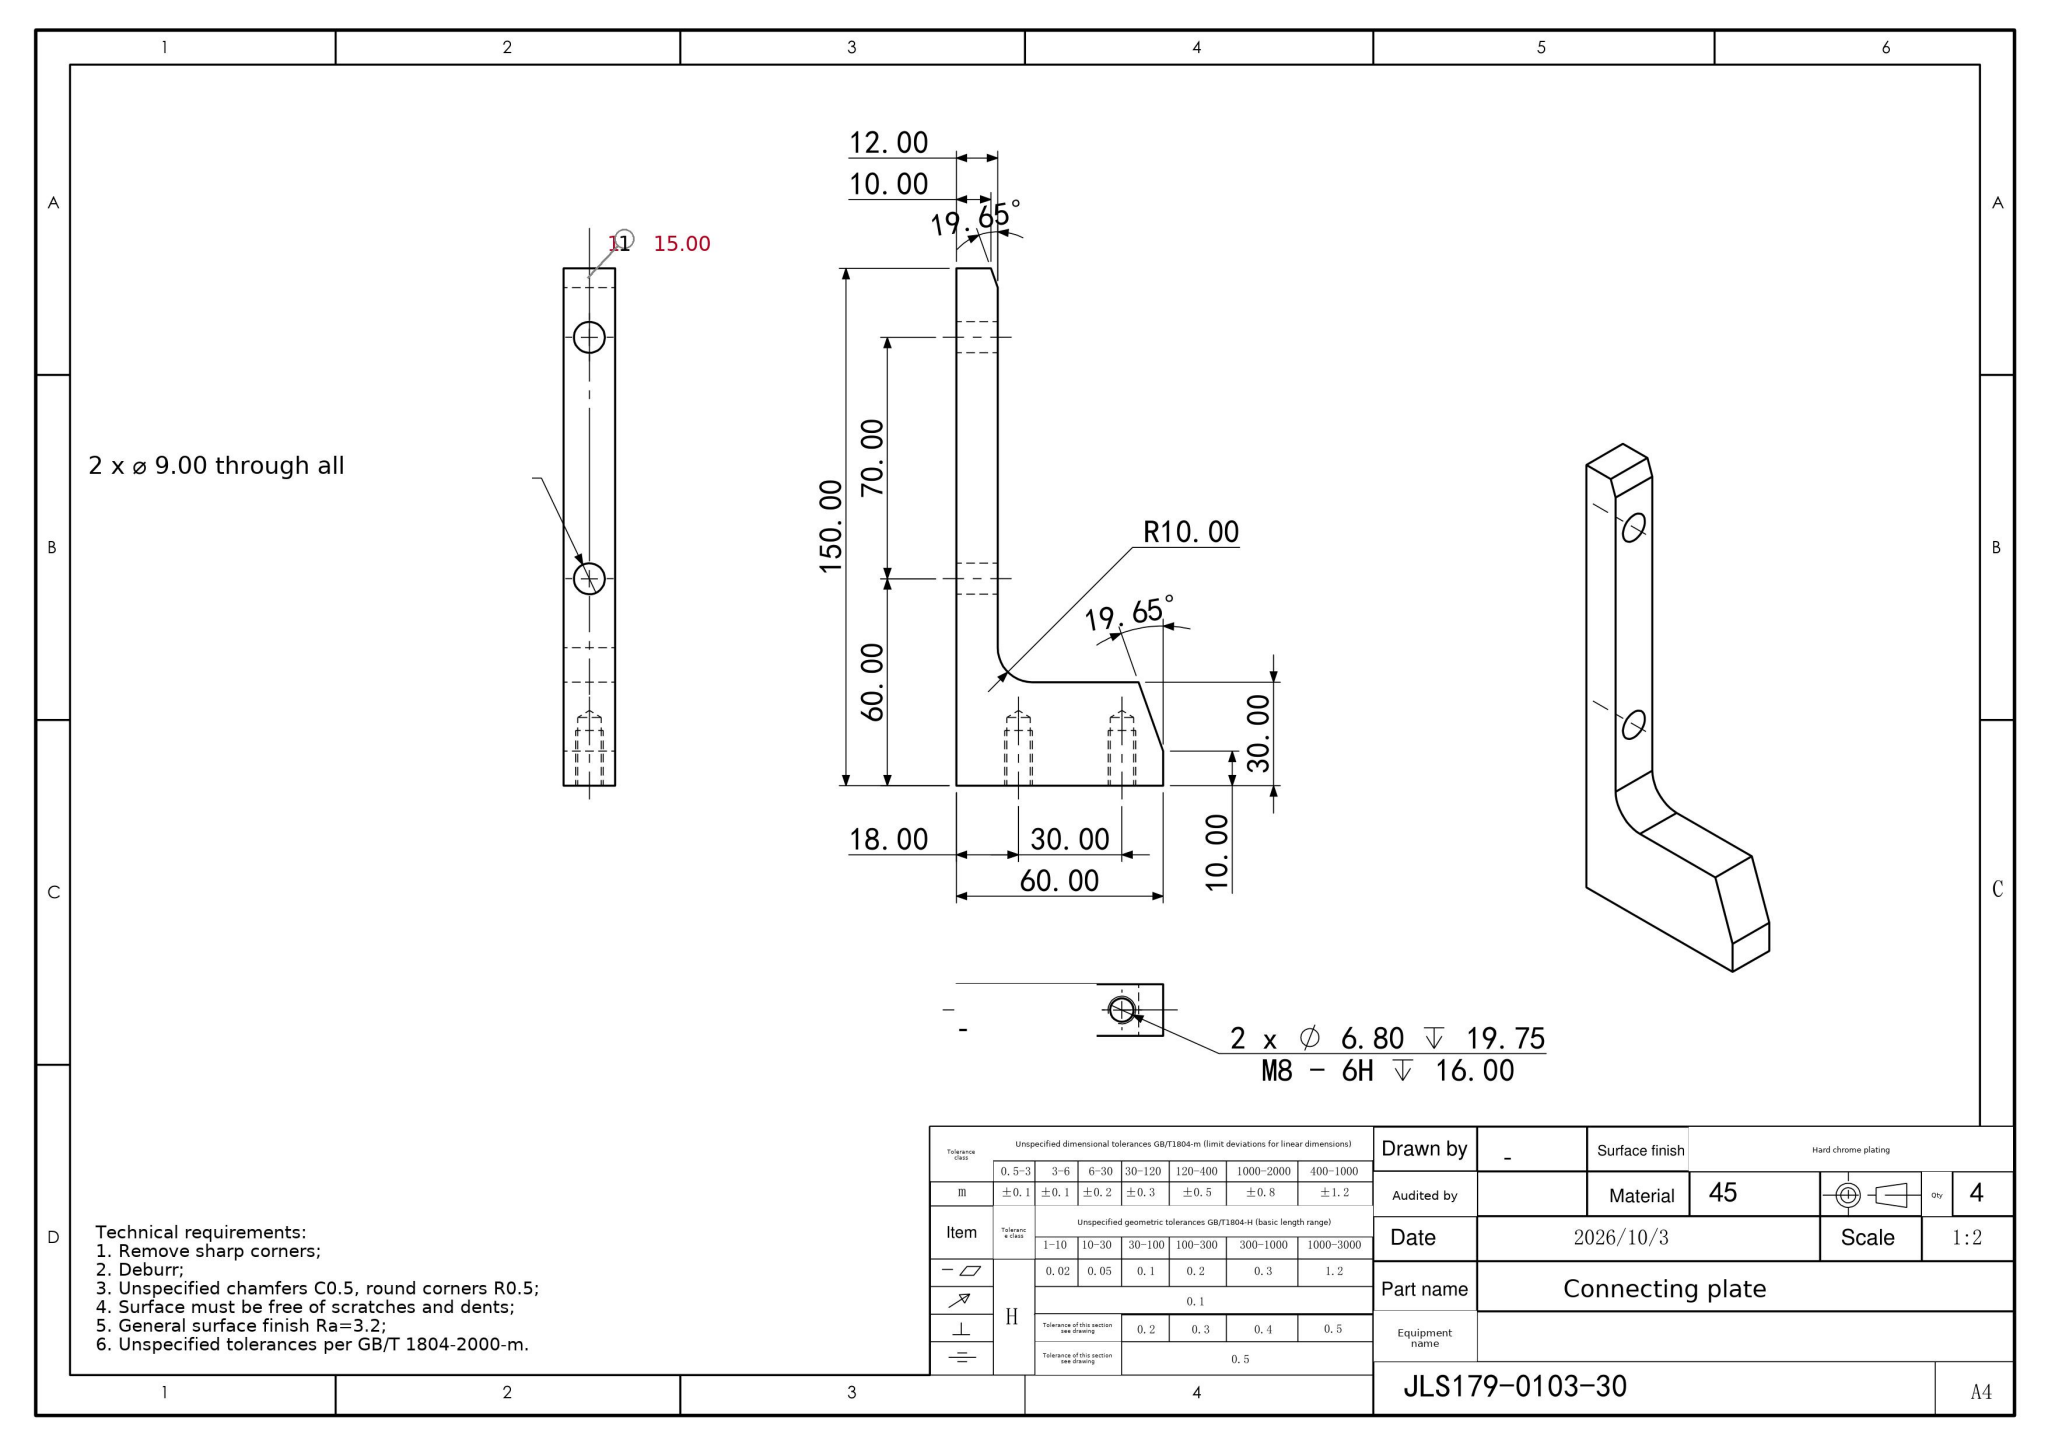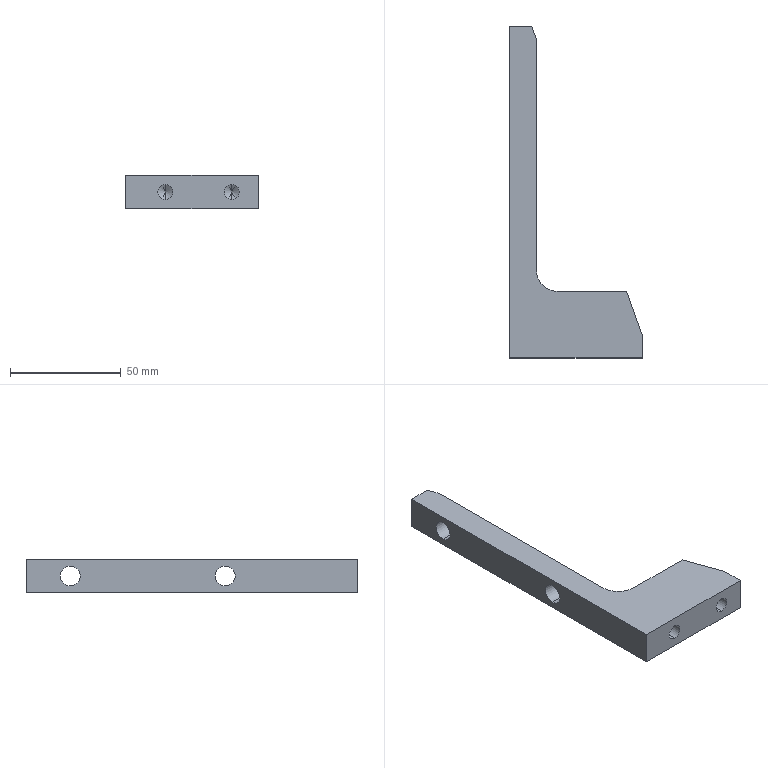Part | SolidWorks | mm | material 45 | 1 solid | 23 faces | box 60 x 150 x 15 mm | volume 44756 mm3 | plane 10 | cylinder 9 | cone 4 | commonest cylinder face diameters 6.8 x4 9 x4 20 x1
build123d program:
from build123d import *

# Parameters (mm, degrees)
BOSS_EXTRUDE1_DEPTH      = 7.5
F_9_0_9_DIAMETER_HOLE1_D = 9
M8_TAPPED_HOLE2_D        = 6.8
M8_TAPPED_HOLE2_DEPTH    = 19.75
M8_TAPPED_HOLE2_TIP      = 2.043
SKETCH6_W                = 90.036
SKETCH6_H                = 126.144
CUT_EXTRUDE1_DEPTH       = 163.25
FILLET1_R                = 10


with BuildPart() as part:
    # Sketch1 → Boss-Extrude1 (new, symmetric)
    with BuildSketch(Plane.XY):
        Polygon((0, 0), (0, 150), (10, 150), (60, 10), (60, 0), align=None)
    extrude(amount=BOSS_EXTRUDE1_DEPTH, both=True)

    # 9.0 _9_ Diameter Hole1 (through all)
    with Locations(Plane.ZY):
        with Locations((0, 130), (0, 60)):
            Hole(F_9_0_9_DIAMETER_HOLE1_D / 2)

    # M8 Tapped Hole2
    with Locations(Plane(origin=(0, 0, 0), x_dir=(-1, 0, 0), z_dir=(0, -1, 0))):
        with Locations((-48, 0), (-18, 0)):
            Hole(M8_TAPPED_HOLE2_D / 2, depth=M8_TAPPED_HOLE2_DEPTH)
            with Locations((0, 0, -(M8_TAPPED_HOLE2_DEPTH + M8_TAPPED_HOLE2_TIP / 2))):  # 118° drill point
                Cone(0, M8_TAPPED_HOLE2_D / 2, M8_TAPPED_HOLE2_TIP, mode=Mode.SUBTRACT)

    # Sketch6 → Cut-Extrude1 (cut, through all)
    with BuildSketch(Plane.XY.offset(7.5)):
        with Locations((57.018, 93.072)):
            Rectangle(SKETCH6_W, SKETCH6_H)
    extrude(amount=-CUT_EXTRUDE1_DEPTH, mode=Mode.SUBTRACT)

    # Fillet1
    fillet1_edges = [part.edges().sort_by_distance(p)[0] for p in [
        (12, 30, 0),
    ]]
    fillet(fillet1_edges, radius=FILLET1_R)


solid = part.part
STEP:
#1=CARTESIAN_POINT('',(48.,19.75,3.4));
#2=VERTEX_POINT('',#1);
#3=CARTESIAN_POINT('',(48.,19.75,-3.4));
#4=VERTEX_POINT('',#3);
#5=CARTESIAN_POINT('',(48.,19.75,0.));
#6=DIRECTION('',(0.,-1.,0.));
#7=DIRECTION('',(0.,0.,-1.));
#8=AXIS2_PLACEMENT_3D('',#5,#6,#7);
#9=CIRCLE('',#8,3.4);
#10=EDGE_CURVE('',#2,#4,#9,.T.);
#11=ORIENTED_EDGE('',*,*,#10,.F.);
#12=CARTESIAN_POINT('',(48.,-0.,3.4));
#13=VERTEX_POINT('',#12);
#14=CARTESIAN_POINT('',(48.,-0.,3.4));
#15=DIRECTION('',(0.,-1.,0.));
#16=VECTOR('',#15,1000.);
#17=LINE('',#14,#16);
#18=EDGE_CURVE('',#2,#13,#17,.T.);
#19=ORIENTED_EDGE('',*,*,#18,.T.);
#20=CARTESIAN_POINT('',(48.,-0.,-3.4));
#21=VERTEX_POINT('',#20);
#22=CARTESIAN_POINT('',(48.,-0.,0.));
#23=DIRECTION('',(0.,-1.,0.));
#24=DIRECTION('',(0.,0.,-1.));
#25=AXIS2_PLACEMENT_3D('',#22,#23,#24);
#26=CIRCLE('',#25,3.4);
#27=EDGE_CURVE('',#13,#21,#26,.T.);
#28=ORIENTED_EDGE('',*,*,#27,.T.);
#29=CARTESIAN_POINT('',(48.,-0.,-3.4));
#30=DIRECTION('',(0.,-1.,0.));
#31=VECTOR('',#30,1000.);
#32=LINE('',#29,#31);
#33=EDGE_CURVE('',#4,#21,#32,.T.);
#34=ORIENTED_EDGE('',*,*,#33,.F.);
#35=EDGE_LOOP('',(#11,#19,#28,#34));
#36=FACE_OUTER_BOUND('',#35,.T.);
#37=CARTESIAN_POINT('',(48.,-0.,0.));
#38=DIRECTION('',(0.,-1.,0.));
#39=DIRECTION('',(0.,0.,-1.));
#40=AXIS2_PLACEMENT_3D('',#37,#38,#39);
#41=CYLINDRICAL_SURFACE('',#40,3.4);
#42=ADVANCED_FACE('',(#36),#41,.F.);
#43=CARTESIAN_POINT('',(48.,21.793,0.));
#44=VERTEX_POINT('',#43);
#45=CARTESIAN_POINT('',(48.,19.75,-3.4));
#46=DIRECTION('',(0.,-0.515,-0.8572));
#47=VECTOR('',#46,1000.);
#48=LINE('',#45,#47);
#49=EDGE_CURVE('',#44,#4,#48,.T.);
#50=ORIENTED_EDGE('',*,*,#49,.F.);
#51=CARTESIAN_POINT('',(48.,19.75,3.4));
#52=DIRECTION('',(0.,-0.515,0.8572));
#53=VECTOR('',#52,1000.);
#54=LINE('',#51,#53);
#55=EDGE_CURVE('',#44,#2,#54,.T.);
#56=ORIENTED_EDGE('',*,*,#55,.T.);
#57=ORIENTED_EDGE('',*,*,#10,.T.);
#58=EDGE_LOOP('',(#50,#56,#57));
#59=FACE_OUTER_BOUND('',#58,.T.);
#60=CARTESIAN_POINT('',(48.,19.75,0.));
#61=DIRECTION('',(0.,-1.,0.));
#62=DIRECTION('',(0.,0.,-1.));
#63=AXIS2_PLACEMENT_3D('',#60,#61,#62);
#64=CONICAL_SURFACE('',#63,3.4,1.03);
#65=ADVANCED_FACE('',(#59),#64,.F.);
#66=CARTESIAN_POINT('',(18.,19.75,3.4));
#67=VERTEX_POINT('',#66);
#68=CARTESIAN_POINT('',(18.,19.75,-3.4));
#69=VERTEX_POINT('',#68);
#70=CARTESIAN_POINT('',(18.,19.75,0.));
#71=DIRECTION('',(0.,-1.,0.));
#72=DIRECTION('',(0.,0.,-1.));
#73=AXIS2_PLACEMENT_3D('',#70,#71,#72);
#74=CIRCLE('',#73,3.4);
#75=EDGE_CURVE('',#67,#69,#74,.T.);
#76=ORIENTED_EDGE('',*,*,#75,.F.);
#77=CARTESIAN_POINT('',(18.,-0.,3.4));
#78=VERTEX_POINT('',#77);
#79=CARTESIAN_POINT('',(18.,-0.,3.4));
#80=DIRECTION('',(0.,-1.,0.));
#81=VECTOR('',#80,1000.);
#82=LINE('',#79,#81);
#83=EDGE_CURVE('',#67,#78,#82,.T.);
#84=ORIENTED_EDGE('',*,*,#83,.T.);
#85=CARTESIAN_POINT('',(18.,-0.,-3.4));
#86=VERTEX_POINT('',#85);
#87=CARTESIAN_POINT('',(18.,-0.,0.));
#88=DIRECTION('',(0.,-1.,0.));
#89=DIRECTION('',(0.,0.,-1.));
#90=AXIS2_PLACEMENT_3D('',#87,#88,#89);
#91=CIRCLE('',#90,3.4);
#92=EDGE_CURVE('',#78,#86,#91,.T.);
#93=ORIENTED_EDGE('',*,*,#92,.T.);
#94=CARTESIAN_POINT('',(18.,-0.,-3.4));
#95=DIRECTION('',(0.,-1.,0.));
#96=VECTOR('',#95,1000.);
#97=LINE('',#94,#96);
#98=EDGE_CURVE('',#69,#86,#97,.T.);
#99=ORIENTED_EDGE('',*,*,#98,.F.);
#100=EDGE_LOOP('',(#76,#84,#93,#99));
#101=FACE_OUTER_BOUND('',#100,.T.);
#102=CARTESIAN_POINT('',(18.,-0.,0.));
#103=DIRECTION('',(0.,-1.,0.));
#104=DIRECTION('',(0.,0.,-1.));
#105=AXIS2_PLACEMENT_3D('',#102,#103,#104);
#106=CYLINDRICAL_SURFACE('',#105,3.4);
#107=ADVANCED_FACE('',(#101),#106,.F.);
#108=CARTESIAN_POINT('',(18.,21.793,0.));
#109=VERTEX_POINT('',#108);
#110=CARTESIAN_POINT('',(18.,19.75,-3.4));
#111=DIRECTION('',(0.,-0.515,-0.8572));
#112=VECTOR('',#111,1000.);
#113=LINE('',#110,#112);
#114=EDGE_CURVE('',#109,#69,#113,.T.);
#115=ORIENTED_EDGE('',*,*,#114,.F.);
#116=CARTESIAN_POINT('',(18.,19.75,3.4));
#117=DIRECTION('',(0.,-0.515,0.8572));
#118=VECTOR('',#117,1000.);
#119=LINE('',#116,#118);
#120=EDGE_CURVE('',#109,#67,#119,.T.);
#121=ORIENTED_EDGE('',*,*,#120,.T.);
#122=ORIENTED_EDGE('',*,*,#75,.T.);
#123=EDGE_LOOP('',(#115,#121,#122));
#124=FACE_OUTER_BOUND('',#123,.T.);
#125=CARTESIAN_POINT('',(18.,19.75,0.));
#126=DIRECTION('',(0.,-1.,0.));
#127=DIRECTION('',(0.,0.,-1.));
#128=AXIS2_PLACEMENT_3D('',#125,#126,#127);
#129=CONICAL_SURFACE('',#128,3.4,1.03);
#130=ADVANCED_FACE('',(#124),#129,.F.);
#131=CARTESIAN_POINT('',(12.,130.,4.5));
#132=VERTEX_POINT('',#131);
#133=CARTESIAN_POINT('',(12.,130.,-4.5));
#134=VERTEX_POINT('',#133);
#135=CARTESIAN_POINT('',(12.,130.,0.));
#136=DIRECTION('',(1.,0.,0.));
#137=DIRECTION('',(0.,-1.,0.));
#138=AXIS2_PLACEMENT_3D('',#135,#136,#137);
#139=CIRCLE('',#138,4.5);
#140=EDGE_CURVE('',#132,#134,#139,.T.);
#141=ORIENTED_EDGE('',*,*,#140,.T.);
#142=CARTESIAN_POINT('',(-0.,130.,-4.5));
#143=VERTEX_POINT('',#142);
#144=CARTESIAN_POINT('',(0.,130.,-4.5));
#145=DIRECTION('',(-1.,0.,0.));
#146=VECTOR('',#145,1000.);
#147=LINE('',#144,#146);
#148=EDGE_CURVE('',#134,#143,#147,.T.);
#149=ORIENTED_EDGE('',*,*,#148,.T.);
#150=CARTESIAN_POINT('',(-0.,130.,4.5));
#151=VERTEX_POINT('',#150);
#152=CARTESIAN_POINT('',(-0.,130.,0.));
#153=DIRECTION('',(-1.,0.,0.));
#154=DIRECTION('',(0.,0.,1.));
#155=AXIS2_PLACEMENT_3D('',#152,#153,#154);
#156=CIRCLE('',#155,4.5);
#157=EDGE_CURVE('',#143,#151,#156,.T.);
#158=ORIENTED_EDGE('',*,*,#157,.T.);
#159=CARTESIAN_POINT('',(0.,130.,4.5));
#160=DIRECTION('',(-1.,0.,0.));
#161=VECTOR('',#160,1000.);
#162=LINE('',#159,#161);
#163=EDGE_CURVE('',#132,#151,#162,.T.);
#164=ORIENTED_EDGE('',*,*,#163,.F.);
#165=EDGE_LOOP('',(#141,#149,#158,#164));
#166=FACE_OUTER_BOUND('',#165,.T.);
#167=CARTESIAN_POINT('',(0.,130.,0.));
#168=DIRECTION('',(-1.,0.,0.));
#169=DIRECTION('',(0.,0.,1.));
#170=AXIS2_PLACEMENT_3D('',#167,#168,#169);
#171=CYLINDRICAL_SURFACE('',#170,4.5);
#172=ADVANCED_FACE('',(#166),#171,.F.);
#173=CARTESIAN_POINT('',(12.,60.,4.5));
#174=VERTEX_POINT('',#173);
#175=CARTESIAN_POINT('',(12.,60.,-4.5));
#176=VERTEX_POINT('',#175);
#177=CARTESIAN_POINT('',(12.,60.,0.));
#178=DIRECTION('',(1.,0.,0.));
#179=DIRECTION('',(0.,-1.,0.));
#180=AXIS2_PLACEMENT_3D('',#177,#178,#179);
#181=CIRCLE('',#180,4.5);
#182=EDGE_CURVE('',#174,#176,#181,.T.);
#183=ORIENTED_EDGE('',*,*,#182,.T.);
#184=CARTESIAN_POINT('',(-0.,60.,-4.5));
#185=VERTEX_POINT('',#184);
#186=CARTESIAN_POINT('',(0.,60.,-4.5));
#187=DIRECTION('',(-1.,0.,0.));
#188=VECTOR('',#187,1000.);
#189=LINE('',#186,#188);
#190=EDGE_CURVE('',#176,#185,#189,.T.);
#191=ORIENTED_EDGE('',*,*,#190,.T.);
#192=CARTESIAN_POINT('',(-0.,60.,4.5));
#193=VERTEX_POINT('',#192);
#194=CARTESIAN_POINT('',(-0.,60.,0.));
#195=DIRECTION('',(-1.,0.,0.));
#196=DIRECTION('',(0.,0.,1.));
#197=AXIS2_PLACEMENT_3D('',#194,#195,#196);
#198=CIRCLE('',#197,4.5);
#199=EDGE_CURVE('',#185,#193,#198,.T.);
#200=ORIENTED_EDGE('',*,*,#199,.T.);
#201=CARTESIAN_POINT('',(0.,60.,4.5));
#202=DIRECTION('',(-1.,0.,0.));
#203=VECTOR('',#202,1000.);
#204=LINE('',#201,#203);
#205=EDGE_CURVE('',#174,#193,#204,.T.);
#206=ORIENTED_EDGE('',*,*,#205,.F.);
#207=EDGE_LOOP('',(#183,#191,#200,#206));
#208=FACE_OUTER_BOUND('',#207,.T.);
#209=CARTESIAN_POINT('',(0.,60.,0.));
#210=DIRECTION('',(-1.,0.,0.));
#211=DIRECTION('',(0.,0.,1.));
#212=AXIS2_PLACEMENT_3D('',#209,#210,#211);
#213=CYLINDRICAL_SURFACE('',#212,4.5);
#214=ADVANCED_FACE('',(#208),#213,.F.);
#215=CARTESIAN_POINT('',(12.,144.4,7.5));
#216=VERTEX_POINT('',#215);
#217=CARTESIAN_POINT('',(10.,150.,7.5));
#218=VERTEX_POINT('',#217);
#219=CARTESIAN_POINT('',(10.,150.,7.5));
#220=DIRECTION('',(-0.3363,0.9417,0.));
#221=VECTOR('',#220,1000.);
#222=LINE('',#219,#221);
#223=EDGE_CURVE('',#216,#218,#222,.T.);
#224=ORIENTED_EDGE('',*,*,#223,.F.);
#225=CARTESIAN_POINT('',(12.,144.4,-7.5));
#226=VERTEX_POINT('',#225);
#227=CARTESIAN_POINT('',(12.,144.4,7.5));
#228=DIRECTION('',(0.,0.,-1.));
#229=VECTOR('',#228,1000.);
#230=LINE('',#227,#229);
#231=EDGE_CURVE('',#216,#226,#230,.T.);
#232=ORIENTED_EDGE('',*,*,#231,.T.);
#233=CARTESIAN_POINT('',(10.,150.,-7.5));
#234=VERTEX_POINT('',#233);
#235=CARTESIAN_POINT('',(10.,150.,-7.5));
#236=DIRECTION('',(-0.3363,0.9417,0.));
#237=VECTOR('',#236,1000.);
#238=LINE('',#235,#237);
#239=EDGE_CURVE('',#226,#234,#238,.T.);
#240=ORIENTED_EDGE('',*,*,#239,.T.);
#241=CARTESIAN_POINT('',(10.,150.,7.5));
#242=DIRECTION('',(0.,0.,-1.));
#243=VECTOR('',#242,1000.);
#244=LINE('',#241,#243);
#245=EDGE_CURVE('',#218,#234,#244,.T.);
#246=ORIENTED_EDGE('',*,*,#245,.F.);
#247=EDGE_LOOP('',(#224,#232,#240,#246));
#248=FACE_OUTER_BOUND('',#247,.T.);
#249=CARTESIAN_POINT('',(10.,150.,7.5));
#250=DIRECTION('',(-0.9417,-0.3363,0.));
#251=DIRECTION('',(0.3363,-0.9417,0.));
#252=AXIS2_PLACEMENT_3D('',#249,#250,#251);
#253=PLANE('',#252);
#254=ADVANCED_FACE('',(#248),#253,.F.);
#255=CARTESIAN_POINT('',(-0.,60.,0.));
#256=DIRECTION('',(-1.,0.,0.));
#257=DIRECTION('',(0.,0.,1.));
#258=AXIS2_PLACEMENT_3D('',#255,#256,#257);
#259=CIRCLE('',#258,4.5);
#260=EDGE_CURVE('',#193,#185,#259,.T.);
#261=ORIENTED_EDGE('',*,*,#260,.F.);
#262=ORIENTED_EDGE('',*,*,#199,.F.);
#263=EDGE_LOOP('',(#261,#262));
#264=FACE_BOUND('',#263,.T.);
#265=CARTESIAN_POINT('',(0.,150.,-7.5));
#266=VERTEX_POINT('',#265);
#267=CARTESIAN_POINT('',(0.,0.,-7.5));
#268=VERTEX_POINT('',#267);
#269=CARTESIAN_POINT('',(0.,0.,-7.5));
#270=DIRECTION('',(0.,-1.,0.));
#271=VECTOR('',#270,1000.);
#272=LINE('',#269,#271);
#273=EDGE_CURVE('',#266,#268,#272,.T.);
#274=ORIENTED_EDGE('',*,*,#273,.T.);
#275=CARTESIAN_POINT('',(0.,0.,7.5));
#276=VERTEX_POINT('',#275);
#277=CARTESIAN_POINT('',(0.,0.,7.5));
#278=DIRECTION('',(0.,0.,-1.));
#279=VECTOR('',#278,1000.);
#280=LINE('',#277,#279);
#281=EDGE_CURVE('',#276,#268,#280,.T.);
#282=ORIENTED_EDGE('',*,*,#281,.F.);
#283=CARTESIAN_POINT('',(0.,150.,7.5));
#284=VERTEX_POINT('',#283);
#285=CARTESIAN_POINT('',(0.,0.,7.5));
#286=DIRECTION('',(0.,-1.,0.));
#287=VECTOR('',#286,1000.);
#288=LINE('',#285,#287);
#289=EDGE_CURVE('',#284,#276,#288,.T.);
#290=ORIENTED_EDGE('',*,*,#289,.F.);
#291=CARTESIAN_POINT('',(0.,150.,7.5));
#292=DIRECTION('',(0.,0.,-1.));
#293=VECTOR('',#292,1000.);
#294=LINE('',#291,#293);
#295=EDGE_CURVE('',#284,#266,#294,.T.);
#296=ORIENTED_EDGE('',*,*,#295,.T.);
#297=EDGE_LOOP('',(#274,#282,#290,#296));
#298=FACE_OUTER_BOUND('',#297,.T.);
#299=CARTESIAN_POINT('',(-0.,130.,0.));
#300=DIRECTION('',(-1.,0.,0.));
#301=DIRECTION('',(0.,0.,1.));
#302=AXIS2_PLACEMENT_3D('',#299,#300,#301);
#303=CIRCLE('',#302,4.5);
#304=EDGE_CURVE('',#151,#143,#303,.T.);
#305=ORIENTED_EDGE('',*,*,#304,.F.);
#306=ORIENTED_EDGE('',*,*,#157,.F.);
#307=EDGE_LOOP('',(#305,#306));
#308=FACE_BOUND('',#307,.T.);
#309=CARTESIAN_POINT('',(0.,0.,7.5));
#310=DIRECTION('',(1.,0.,0.));
#311=DIRECTION('',(0.,0.,-1.));
#312=AXIS2_PLACEMENT_3D('',#309,#310,#311);
#313=PLANE('',#312);
#314=ADVANCED_FACE('',(#264,#298,#308),#313,.F.);
#315=CARTESIAN_POINT('',(48.,-0.,0.));
#316=DIRECTION('',(0.,-1.,0.));
#317=DIRECTION('',(0.,0.,-1.));
#318=AXIS2_PLACEMENT_3D('',#315,#316,#317);
#319=CIRCLE('',#318,3.4);
#320=EDGE_CURVE('',#21,#13,#319,.T.);
#321=ORIENTED_EDGE('',*,*,#320,.F.);
#322=ORIENTED_EDGE('',*,*,#27,.F.);
#323=EDGE_LOOP('',(#321,#322));
#324=FACE_BOUND('',#323,.T.);
#325=CARTESIAN_POINT('',(18.,-0.,0.));
#326=DIRECTION('',(0.,-1.,0.));
#327=DIRECTION('',(0.,0.,-1.));
#328=AXIS2_PLACEMENT_3D('',#325,#326,#327);
#329=CIRCLE('',#328,3.4);
#330=EDGE_CURVE('',#86,#78,#329,.T.);
#331=ORIENTED_EDGE('',*,*,#330,.F.);
#332=ORIENTED_EDGE('',*,*,#92,.F.);
#333=EDGE_LOOP('',(#331,#332));
#334=FACE_BOUND('',#333,.T.);
#335=CARTESIAN_POINT('',(60.,-0.,-7.5));
#336=VERTEX_POINT('',#335);
#337=CARTESIAN_POINT('',(60.,-0.,-7.5));
#338=DIRECTION('',(1.,-0.,0.));
#339=VECTOR('',#338,1000.);
#340=LINE('',#337,#339);
#341=EDGE_CURVE('',#268,#336,#340,.T.);
#342=ORIENTED_EDGE('',*,*,#341,.T.);
#343=CARTESIAN_POINT('',(60.,-0.,7.5));
#344=VERTEX_POINT('',#343);
#345=CARTESIAN_POINT('',(60.,-0.,7.5));
#346=DIRECTION('',(0.,0.,-1.));
#347=VECTOR('',#346,1000.);
#348=LINE('',#345,#347);
#349=EDGE_CURVE('',#344,#336,#348,.T.);
#350=ORIENTED_EDGE('',*,*,#349,.F.);
#351=CARTESIAN_POINT('',(60.,-0.,7.5));
#352=DIRECTION('',(1.,-0.,0.));
#353=VECTOR('',#352,1000.);
#354=LINE('',#351,#353);
#355=EDGE_CURVE('',#276,#344,#354,.T.);
#356=ORIENTED_EDGE('',*,*,#355,.F.);
#357=ORIENTED_EDGE('',*,*,#281,.T.);
#358=EDGE_LOOP('',(#342,#350,#356,#357));
#359=FACE_OUTER_BOUND('',#358,.T.);
#360=CARTESIAN_POINT('',(60.,-0.,7.5));
#361=DIRECTION('',(0.,1.,0.));
#362=DIRECTION('',(-1.,0.,0.));
#363=AXIS2_PLACEMENT_3D('',#360,#361,#362);
#364=PLANE('',#363);
#365=ADVANCED_FACE('',(#324,#334,#359),#364,.F.);
#366=CARTESIAN_POINT('',(60.,10.,-7.5));
#367=VERTEX_POINT('',#366);
#368=CARTESIAN_POINT('',(60.,10.,-7.5));
#369=DIRECTION('',(0.,1.,0.));
#370=VECTOR('',#369,1000.);
#371=LINE('',#368,#370);
#372=EDGE_CURVE('',#336,#367,#371,.T.);
#373=ORIENTED_EDGE('',*,*,#372,.T.);
#374=CARTESIAN_POINT('',(60.,10.,7.5));
#375=VERTEX_POINT('',#374);
#376=CARTESIAN_POINT('',(60.,10.,7.5));
#377=DIRECTION('',(0.,0.,-1.));
#378=VECTOR('',#377,1000.);
#379=LINE('',#376,#378);
#380=EDGE_CURVE('',#375,#367,#379,.T.);
#381=ORIENTED_EDGE('',*,*,#380,.F.);
#382=CARTESIAN_POINT('',(60.,10.,7.5));
#383=DIRECTION('',(0.,1.,0.));
#384=VECTOR('',#383,1000.);
#385=LINE('',#382,#384);
#386=EDGE_CURVE('',#344,#375,#385,.T.);
#387=ORIENTED_EDGE('',*,*,#386,.F.);
#388=ORIENTED_EDGE('',*,*,#349,.T.);
#389=EDGE_LOOP('',(#373,#381,#387,#388));
#390=FACE_OUTER_BOUND('',#389,.T.);
#391=CARTESIAN_POINT('',(60.,10.,7.5));
#392=DIRECTION('',(-1.,0.,0.));
#393=DIRECTION('',(0.,0.,1.));
#394=AXIS2_PLACEMENT_3D('',#391,#392,#393);
#395=PLANE('',#394);
#396=ADVANCED_FACE('',(#390),#395,.F.);
#397=CARTESIAN_POINT('',(52.857,30.,-7.5));
#398=VERTEX_POINT('',#397);
#399=CARTESIAN_POINT('',(10.,150.,-7.5));
#400=DIRECTION('',(-0.3363,0.9417,0.));
#401=VECTOR('',#400,1000.);
#402=LINE('',#399,#401);
#403=EDGE_CURVE('',#367,#398,#402,.T.);
#404=ORIENTED_EDGE('',*,*,#403,.T.);
#405=CARTESIAN_POINT('',(52.857,30.,7.5));
#406=VERTEX_POINT('',#405);
#407=CARTESIAN_POINT('',(52.857,30.,7.5));
#408=DIRECTION('',(0.,0.,1.));
#409=VECTOR('',#408,1000.);
#410=LINE('',#407,#409);
#411=EDGE_CURVE('',#398,#406,#410,.T.);
#412=ORIENTED_EDGE('',*,*,#411,.T.);
#413=CARTESIAN_POINT('',(10.,150.,7.5));
#414=DIRECTION('',(-0.3363,0.9417,0.));
#415=VECTOR('',#414,1000.);
#416=LINE('',#413,#415);
#417=EDGE_CURVE('',#375,#406,#416,.T.);
#418=ORIENTED_EDGE('',*,*,#417,.F.);
#419=ORIENTED_EDGE('',*,*,#380,.T.);
#420=EDGE_LOOP('',(#404,#412,#418,#419));
#421=FACE_OUTER_BOUND('',#420,.T.);
#422=CARTESIAN_POINT('',(10.,150.,7.5));
#423=DIRECTION('',(-0.9417,-0.3363,0.));
#424=DIRECTION('',(0.3363,-0.9417,0.));
#425=AXIS2_PLACEMENT_3D('',#422,#423,#424);
#426=PLANE('',#425);
#427=ADVANCED_FACE('',(#421),#426,.F.);
#428=CARTESIAN_POINT('',(0.,150.,-7.5));
#429=DIRECTION('',(-1.,0.,0.));
#430=VECTOR('',#429,1000.);
#431=LINE('',#428,#430);
#432=EDGE_CURVE('',#234,#266,#431,.T.);
#433=ORIENTED_EDGE('',*,*,#432,.T.);
#434=ORIENTED_EDGE('',*,*,#295,.F.);
#435=CARTESIAN_POINT('',(0.,150.,7.5));
#436=DIRECTION('',(-1.,0.,0.));
#437=VECTOR('',#436,1000.);
#438=LINE('',#435,#437);
#439=EDGE_CURVE('',#218,#284,#438,.T.);
#440=ORIENTED_EDGE('',*,*,#439,.F.);
#441=ORIENTED_EDGE('',*,*,#245,.T.);
#442=EDGE_LOOP('',(#433,#434,#440,#441));
#443=FACE_OUTER_BOUND('',#442,.T.);
#444=CARTESIAN_POINT('',(0.,150.,7.5));
#445=DIRECTION('',(0.,-1.,0.));
#446=DIRECTION('',(0.,0.,-1.));
#447=AXIS2_PLACEMENT_3D('',#444,#445,#446);
#448=PLANE('',#447);
#449=ADVANCED_FACE('',(#443),#448,.F.);
#450=CARTESIAN_POINT('',(22.,30.,7.5));
#451=VERTEX_POINT('',#450);
#452=CARTESIAN_POINT('',(102.036,30.,7.5));
#453=DIRECTION('',(1.,0.,0.));
#454=VECTOR('',#453,1000.);
#455=LINE('',#452,#454);
#456=EDGE_CURVE('',#451,#406,#455,.T.);
#457=ORIENTED_EDGE('',*,*,#456,.F.);
#458=CARTESIAN_POINT('',(12.,40.,7.5));
#459=VERTEX_POINT('',#458);
#460=CARTESIAN_POINT('',(22.,40.,7.5));
#461=DIRECTION('',(0.,0.,-1.));
#462=DIRECTION('',(-1.,0.,0.));
#463=AXIS2_PLACEMENT_3D('',#460,#461,#462);
#464=CIRCLE('',#463,10.);
#465=EDGE_CURVE('',#451,#459,#464,.T.);
#466=ORIENTED_EDGE('',*,*,#465,.T.);
#467=CARTESIAN_POINT('',(12.,156.144,7.5));
#468=DIRECTION('',(0.,-1.,0.));
#469=VECTOR('',#468,1000.);
#470=LINE('',#467,#469);
#471=EDGE_CURVE('',#216,#459,#470,.T.);
#472=ORIENTED_EDGE('',*,*,#471,.F.);
#473=ORIENTED_EDGE('',*,*,#223,.T.);
#474=ORIENTED_EDGE('',*,*,#439,.T.);
#475=ORIENTED_EDGE('',*,*,#289,.T.);
#476=ORIENTED_EDGE('',*,*,#355,.T.);
#477=ORIENTED_EDGE('',*,*,#386,.T.);
#478=ORIENTED_EDGE('',*,*,#417,.T.);
#479=EDGE_LOOP('',(#457,#466,#472,#473,#474,#475,#476,#477,#478));
#480=FACE_OUTER_BOUND('',#479,.T.);
#481=CARTESIAN_POINT('',(0.,0.,7.5));
#482=DIRECTION('',(0.,0.,-1.));
#483=DIRECTION('',(-1.,0.,0.));
#484=AXIS2_PLACEMENT_3D('',#481,#482,#483);
#485=PLANE('',#484);
#486=ADVANCED_FACE('',(#480),#485,.F.);
#487=CARTESIAN_POINT('',(12.,40.,-7.5));
#488=VERTEX_POINT('',#487);
#489=CARTESIAN_POINT('',(12.,156.144,-7.5));
#490=DIRECTION('',(0.,-1.,0.));
#491=VECTOR('',#490,1000.);
#492=LINE('',#489,#491);
#493=EDGE_CURVE('',#226,#488,#492,.T.);
#494=ORIENTED_EDGE('',*,*,#493,.T.);
#495=CARTESIAN_POINT('',(22.,30.,-7.5));
#496=VERTEX_POINT('',#495);
#497=CARTESIAN_POINT('',(22.,40.,-7.5));
#498=DIRECTION('',(0.,0.,1.));
#499=DIRECTION('',(-1.,-0.,0.));
#500=AXIS2_PLACEMENT_3D('',#497,#498,#499);
#501=CIRCLE('',#500,10.);
#502=EDGE_CURVE('',#488,#496,#501,.T.);
#503=ORIENTED_EDGE('',*,*,#502,.T.);
#504=CARTESIAN_POINT('',(102.036,30.,-7.5));
#505=DIRECTION('',(1.,0.,0.));
#506=VECTOR('',#505,1000.);
#507=LINE('',#504,#506);
#508=EDGE_CURVE('',#496,#398,#507,.T.);
#509=ORIENTED_EDGE('',*,*,#508,.T.);
#510=ORIENTED_EDGE('',*,*,#403,.F.);
#511=ORIENTED_EDGE('',*,*,#372,.F.);
#512=ORIENTED_EDGE('',*,*,#341,.F.);
#513=ORIENTED_EDGE('',*,*,#273,.F.);
#514=ORIENTED_EDGE('',*,*,#432,.F.);
#515=ORIENTED_EDGE('',*,*,#239,.F.);
#516=EDGE_LOOP('',(#494,#503,#509,#510,#511,#512,#513,#514,#515));
#517=FACE_OUTER_BOUND('',#516,.T.);
#518=CARTESIAN_POINT('',(0.,0.,-7.5));
#519=DIRECTION('',(0.,0.,-1.));
#520=DIRECTION('',(-1.,0.,0.));
#521=AXIS2_PLACEMENT_3D('',#518,#519,#520);
#522=PLANE('',#521);
#523=ADVANCED_FACE('',(#517),#522,.T.);
#524=ORIENTED_EDGE('',*,*,#190,.F.);
#525=CARTESIAN_POINT('',(12.,60.,0.));
#526=DIRECTION('',(1.,0.,0.));
#527=DIRECTION('',(0.,-1.,0.));
#528=AXIS2_PLACEMENT_3D('',#525,#526,#527);
#529=CIRCLE('',#528,4.5);
#530=EDGE_CURVE('',#176,#174,#529,.T.);
#531=ORIENTED_EDGE('',*,*,#530,.T.);
#532=ORIENTED_EDGE('',*,*,#205,.T.);
#533=ORIENTED_EDGE('',*,*,#260,.T.);
#534=EDGE_LOOP('',(#524,#531,#532,#533));
#535=FACE_OUTER_BOUND('',#534,.T.);
#536=CARTESIAN_POINT('',(0.,60.,0.));
#537=DIRECTION('',(-1.,0.,0.));
#538=DIRECTION('',(0.,0.,1.));
#539=AXIS2_PLACEMENT_3D('',#536,#537,#538);
#540=CYLINDRICAL_SURFACE('',#539,4.5);
#541=ADVANCED_FACE('',(#535),#540,.F.);
#542=ORIENTED_EDGE('',*,*,#148,.F.);
#543=CARTESIAN_POINT('',(12.,130.,0.));
#544=DIRECTION('',(1.,0.,0.));
#545=DIRECTION('',(0.,-1.,0.));
#546=AXIS2_PLACEMENT_3D('',#543,#544,#545);
#547=CIRCLE('',#546,4.5);
#548=EDGE_CURVE('',#134,#132,#547,.T.);
#549=ORIENTED_EDGE('',*,*,#548,.T.);
#550=ORIENTED_EDGE('',*,*,#163,.T.);
#551=ORIENTED_EDGE('',*,*,#304,.T.);
#552=EDGE_LOOP('',(#542,#549,#550,#551));
#553=FACE_OUTER_BOUND('',#552,.T.);
#554=CARTESIAN_POINT('',(0.,130.,0.));
#555=DIRECTION('',(-1.,0.,0.));
#556=DIRECTION('',(0.,0.,1.));
#557=AXIS2_PLACEMENT_3D('',#554,#555,#556);
#558=CYLINDRICAL_SURFACE('',#557,4.5);
#559=ADVANCED_FACE('',(#553),#558,.F.);
#560=ORIENTED_EDGE('',*,*,#120,.F.);
#561=ORIENTED_EDGE('',*,*,#114,.T.);
#562=CARTESIAN_POINT('',(18.,19.75,0.));
#563=DIRECTION('',(0.,-1.,0.));
#564=DIRECTION('',(0.,0.,-1.));
#565=AXIS2_PLACEMENT_3D('',#562,#563,#564);
#566=CIRCLE('',#565,3.4);
#567=EDGE_CURVE('',#69,#67,#566,.T.);
#568=ORIENTED_EDGE('',*,*,#567,.T.);
#569=EDGE_LOOP('',(#560,#561,#568));
#570=FACE_OUTER_BOUND('',#569,.T.);
#571=CARTESIAN_POINT('',(18.,19.75,0.));
#572=DIRECTION('',(0.,-1.,0.));
#573=DIRECTION('',(0.,0.,-1.));
#574=AXIS2_PLACEMENT_3D('',#571,#572,#573);
#575=CONICAL_SURFACE('',#574,3.4,1.03);
#576=ADVANCED_FACE('',(#570),#575,.F.);
#577=ORIENTED_EDGE('',*,*,#83,.F.);
#578=ORIENTED_EDGE('',*,*,#567,.F.);
#579=ORIENTED_EDGE('',*,*,#98,.T.);
#580=ORIENTED_EDGE('',*,*,#330,.T.);
#581=EDGE_LOOP('',(#577,#578,#579,#580));
#582=FACE_OUTER_BOUND('',#581,.T.);
#583=CARTESIAN_POINT('',(18.,-0.,0.));
#584=DIRECTION('',(0.,-1.,0.));
#585=DIRECTION('',(0.,0.,-1.));
#586=AXIS2_PLACEMENT_3D('',#583,#584,#585);
#587=CYLINDRICAL_SURFACE('',#586,3.4);
#588=ADVANCED_FACE('',(#582),#587,.F.);
#589=ORIENTED_EDGE('',*,*,#55,.F.);
#590=ORIENTED_EDGE('',*,*,#49,.T.);
#591=CARTESIAN_POINT('',(48.,19.75,0.));
#592=DIRECTION('',(0.,-1.,0.));
#593=DIRECTION('',(0.,0.,-1.));
#594=AXIS2_PLACEMENT_3D('',#591,#592,#593);
#595=CIRCLE('',#594,3.4);
#596=EDGE_CURVE('',#4,#2,#595,.T.);
#597=ORIENTED_EDGE('',*,*,#596,.T.);
#598=EDGE_LOOP('',(#589,#590,#597));
#599=FACE_OUTER_BOUND('',#598,.T.);
#600=CARTESIAN_POINT('',(48.,19.75,0.));
#601=DIRECTION('',(0.,-1.,0.));
#602=DIRECTION('',(0.,0.,-1.));
#603=AXIS2_PLACEMENT_3D('',#600,#601,#602);
#604=CONICAL_SURFACE('',#603,3.4,1.03);
#605=ADVANCED_FACE('',(#599),#604,.F.);
#606=ORIENTED_EDGE('',*,*,#18,.F.);
#607=ORIENTED_EDGE('',*,*,#596,.F.);
#608=ORIENTED_EDGE('',*,*,#33,.T.);
#609=ORIENTED_EDGE('',*,*,#320,.T.);
#610=EDGE_LOOP('',(#606,#607,#608,#609));
#611=FACE_OUTER_BOUND('',#610,.T.);
#612=CARTESIAN_POINT('',(48.,-0.,0.));
#613=DIRECTION('',(0.,-1.,0.));
#614=DIRECTION('',(0.,0.,-1.));
#615=AXIS2_PLACEMENT_3D('',#612,#613,#614);
#616=CYLINDRICAL_SURFACE('',#615,3.4);
#617=ADVANCED_FACE('',(#611),#616,.F.);
#618=ORIENTED_EDGE('',*,*,#508,.F.);
#619=CARTESIAN_POINT('',(22.,30.,7.5));
#620=DIRECTION('',(0.,0.,1.));
#621=VECTOR('',#620,1000.);
#622=LINE('',#619,#621);
#623=EDGE_CURVE('',#496,#451,#622,.T.);
#624=ORIENTED_EDGE('',*,*,#623,.T.);
#625=ORIENTED_EDGE('',*,*,#456,.T.);
#626=ORIENTED_EDGE('',*,*,#411,.F.);
#627=EDGE_LOOP('',(#618,#624,#625,#626));
#628=FACE_OUTER_BOUND('',#627,.T.);
#629=CARTESIAN_POINT('',(102.036,30.,-7.5));
#630=DIRECTION('',(0.,-1.,0.));
#631=DIRECTION('',(1.,0.,0.));
#632=AXIS2_PLACEMENT_3D('',#629,#630,#631);
#633=PLANE('',#632);
#634=ADVANCED_FACE('',(#628),#633,.F.);
#635=ORIENTED_EDGE('',*,*,#140,.F.);
#636=ORIENTED_EDGE('',*,*,#548,.F.);
#637=EDGE_LOOP('',(#635,#636));
#638=FACE_BOUND('',#637,.T.);
#639=ORIENTED_EDGE('',*,*,#182,.F.);
#640=ORIENTED_EDGE('',*,*,#530,.F.);
#641=EDGE_LOOP('',(#639,#640));
#642=FACE_BOUND('',#641,.T.);
#643=ORIENTED_EDGE('',*,*,#471,.T.);
#644=CARTESIAN_POINT('',(12.,40.,-7.5));
#645=DIRECTION('',(0.,0.,-1.));
#646=VECTOR('',#645,1000.);
#647=LINE('',#644,#646);
#648=EDGE_CURVE('',#459,#488,#647,.T.);
#649=ORIENTED_EDGE('',*,*,#648,.T.);
#650=ORIENTED_EDGE('',*,*,#493,.F.);
#651=ORIENTED_EDGE('',*,*,#231,.F.);
#652=EDGE_LOOP('',(#643,#649,#650,#651));
#653=FACE_OUTER_BOUND('',#652,.T.);
#654=CARTESIAN_POINT('',(12.,156.144,-7.5));
#655=DIRECTION('',(-1.,-0.,0.));
#656=DIRECTION('',(0.,-1.,0.));
#657=AXIS2_PLACEMENT_3D('',#654,#655,#656);
#658=PLANE('',#657);
#659=ADVANCED_FACE('',(#638,#642,#653),#658,.F.);
#660=ORIENTED_EDGE('',*,*,#502,.F.);
#661=ORIENTED_EDGE('',*,*,#648,.F.);
#662=ORIENTED_EDGE('',*,*,#465,.F.);
#663=ORIENTED_EDGE('',*,*,#623,.F.);
#664=EDGE_LOOP('',(#660,#661,#662,#663));
#665=FACE_OUTER_BOUND('',#664,.T.);
#666=CARTESIAN_POINT('',(22.,40.,-7.5));
#667=DIRECTION('',(0.,0.,-1.));
#668=DIRECTION('',(-1.,0.,0.));
#669=AXIS2_PLACEMENT_3D('',#666,#667,#668);
#670=CYLINDRICAL_SURFACE('',#669,10.);
#671=ADVANCED_FACE('',(#665),#670,.F.);
#672=CLOSED_SHELL('',(#42,#65,#107,#130,#172,#214,#254,#314,#365,#396,#427,#449,#486,#523,#541,#559,#576,#588,#605,#617,#634,#659,#671));
#673=MANIFOLD_SOLID_BREP('',#672);
#674=CARTESIAN_POINT('',(0.,0.,0.));
#675=DIRECTION('',(0.,0.,1.));
#676=DIRECTION('',(1.,0.,0.));
#677=AXIS2_PLACEMENT_3D('',#674,#675,#676);
#678=(LENGTH_UNIT()NAMED_UNIT(*)SI_UNIT(.MILLI.,.METRE.));
#679=UNCERTAINTY_MEASURE_WITH_UNIT(LENGTH_MEASURE(0.00001),#678,'','');
#680=(NAMED_UNIT(*)PLANE_ANGLE_UNIT()SI_UNIT($,.RADIAN.));
#681=(NAMED_UNIT(*)SI_UNIT($,.STERADIAN.)SOLID_ANGLE_UNIT());
#682=(GEOMETRIC_REPRESENTATION_CONTEXT(3)GLOBAL_UNCERTAINTY_ASSIGNED_CONTEXT((#679))GLOBAL_UNIT_ASSIGNED_CONTEXT((#678,#680,#681))REPRESENTATION_CONTEXT('',''));
#683=ADVANCED_BREP_SHAPE_REPRESENTATION('',(#673,#677),#682);